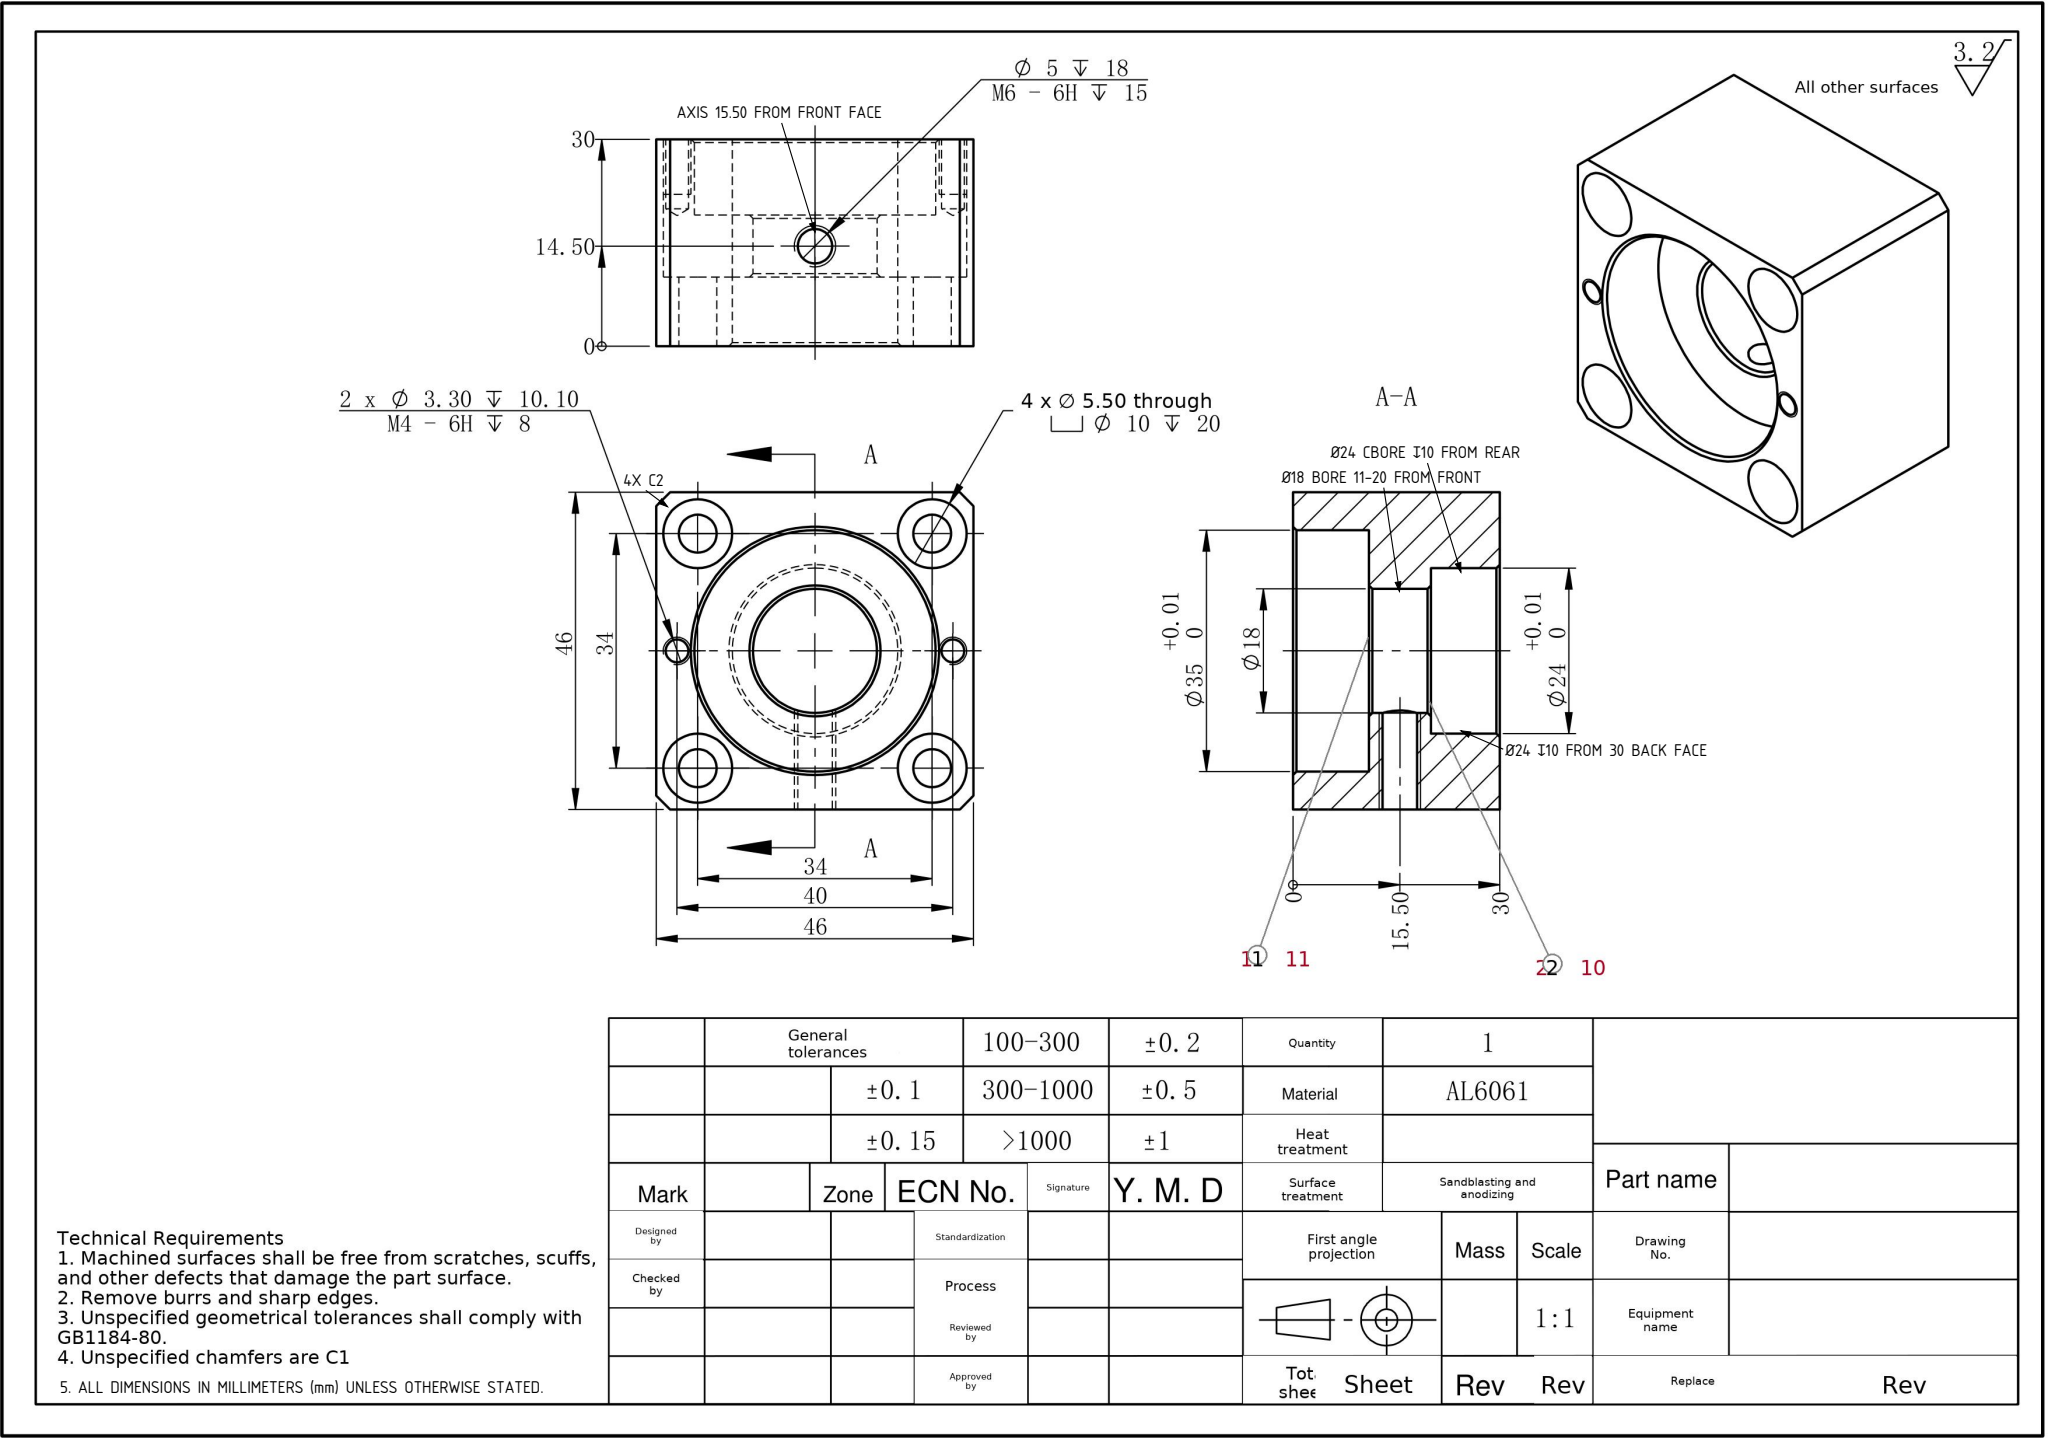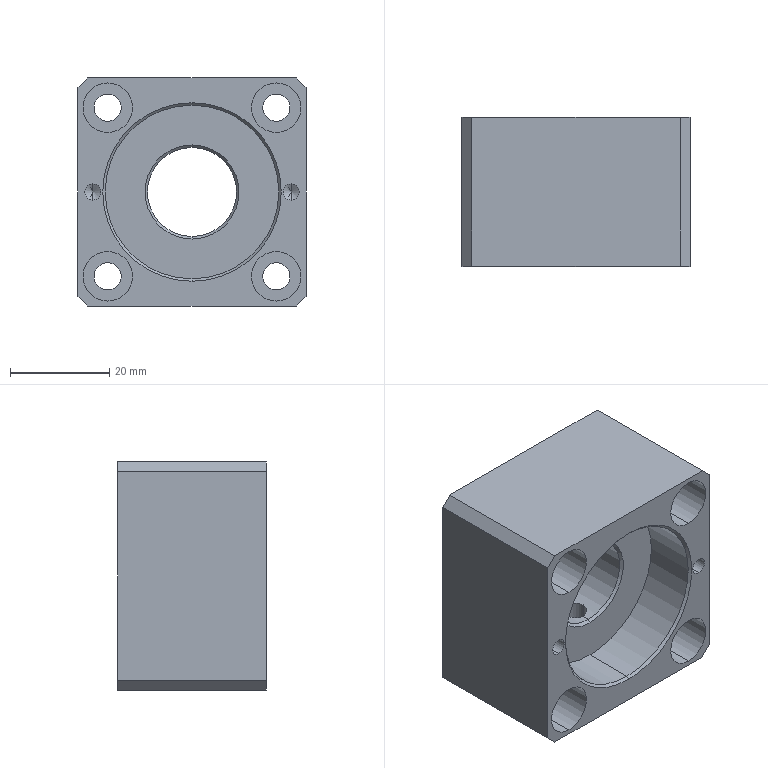Part | SolidWorks | mm | material AL6061 | 1 solid | 56 faces | box 46 x 30 x 46 mm | volume 38116 mm3 | cylinder 28 | plane 16 | cone 12 | commonest cylinder face diameters 10 x8 5.5 x8 3.3 x4 5 x2 35 x2 24 x2 18 x2
Drawing notes:
ALL DIMENSIONS IN MILLIMETERS (mm) UNLESS OTHERWISE STATED. | from the solid: STEP header units mm; bbox_xyz [46.0, 30.0, 46.0]
Ø18 THROUGH-BORE BETWEEN COUNTERBORES, SPANS 11 TO 20 FROM FRONT FACE (Y=0), AXIS AT X=23, Z=23. | from the solid: cylinders: hole/bore Ø18, axis y at [23,null,23], from 11.5 to 19.5 with 90° chamfers at both ends
Ø24 COUNTERBORE, DEPTH 10 FROM REAR FACE (Y=30), COAXIAL WITH Ø18 BORE. | from the solid: cylinders: hole/bore Ø24, axis y at [23,null,23], from 20.0 to 29.5 (0.5 chamfer at mouth)
4X CORNER CHAMFER C2 (2x2x45 DEG) FULL 30 HT, NOT C1 | from the solid: 4 inclined planes 45/90/45 deg, size 2.0 x 30.0 x 2.0 at bbox corners [0,0,0],[0,0,44],[44,0,0],[44,0,44]
M6 HOLE AXIS 15.50 FROM FRONT FACE (0); 14.50 IN TOP VIEW VOID | from the solid: Ø5 bore, axis Z, at [x=23, y=15.5], from z=0 to 14.4
A-A: Ø24 C'BORE DP 10 FROM 30 BACK FACE; '22' VOID | from the solid: Ø24 bore axis Y from y=20.0 to 30.0 (29.5 + 90 deg cone to face y=30), depth 10
build123d program:
from build123d import *

# Parameters (mm, degrees)
SKETCH1_W                                       = 46
SKETCH1_H                                       = 46
BOSS_EXTRUDE1_DEPTH                             = 15
SKETCH4_R                                       = 9
CUT_EXTRUDE1_DEPTH                              = 29
SKETCH5_R                                       = 12
CUT_EXTRUDE2_DEPTH                              = 10
CHAMFER1_SIZE                                   = 2
M5_HEX_SOCKET_HEAD_CAP_SCREW_CBORE1_D           = 5.5
M5_HEX_SOCKET_HEAD_CAP_SCREW_CBORE1_CBORE_D     = 10
M5_HEX_SOCKET_HEAD_CAP_SCREW_CBORE1_CBORE_DEPTH = 20
SKETCH8_R                                       = 17.5
CUT_EXTRUDE3_DEPTH                              = 11
CHAMFER2_SIZE                                   = 0.5
M6_TAPPED_HOLE1_D                               = 5
M6_TAPPED_HOLE1_DEPTH                           = 18
M6_TAPPED_HOLE1_TIP                             = 1.502
M4_TAPPED_HOLE1_D                               = 3.3
M4_TAPPED_HOLE1_DEPTH                           = 10.1
M4_TAPPED_HOLE1_TIP                             = 0.9914


with BuildPart() as part:
    # Sketch1 → Boss-Extrude1 (new, symmetric)
    with BuildSketch(Plane(origin=(0, 0, 0), x_dir=(1, 0, 0), z_dir=(0, 1, 0))):
        Rectangle(SKETCH1_W, SKETCH1_H)
    extrude(amount=BOSS_EXTRUDE1_DEPTH, both=True)

    # Sketch4 → Cut-Extrude1 (cut)
    with BuildSketch(Plane(origin=(0, 15, 0), x_dir=(1, 0, 0), z_dir=(0, 1, 0))):
        with Locations(Location((0, 0, 0), (0, 0, 270))):
            Circle(SKETCH4_R)
    extrude(amount=-CUT_EXTRUDE1_DEPTH, mode=Mode.SUBTRACT)

    # Sketch5 → Cut-Extrude2 (cut)
    with BuildSketch(Plane(origin=(0, 15, 0), x_dir=(1, 0, 0), z_dir=(0, 1, 0))):
        with Locations(Location((0, 0, 0), (0, 0, 270))):
            Circle(SKETCH5_R)
    extrude(amount=-CUT_EXTRUDE2_DEPTH, mode=Mode.SUBTRACT)

    # Chamfer1
    chamfer1_edges = [part.edges().sort_by_distance(p)[0] for p in [
        (23, 0, 23),
        (-23, 0, 23),
        (-23, 0, -23),
        (23, 0, -23),
    ]]
    chamfer(chamfer1_edges, length=CHAMFER1_SIZE)

    # M5 Hex Socket Head Cap Screw CBORE1 (through all)
    with Locations(Plane(origin=(0, -15, 0), x_dir=(-1, 0, 0), z_dir=(0, -1, 0))):
        with Locations((-17, -17), (17, -17), (17, 17), (-17, 17)):
            CounterBoreHole(M5_HEX_SOCKET_HEAD_CAP_SCREW_CBORE1_D / 2, M5_HEX_SOCKET_HEAD_CAP_SCREW_CBORE1_CBORE_D / 2, M5_HEX_SOCKET_HEAD_CAP_SCREW_CBORE1_CBORE_DEPTH)

    # Sketch8 → Cut-Extrude3 (cut)
    with BuildSketch(Plane.XZ.offset(15)):
        with Locations(Location((0, 0, 0), (0, 0, 270))):
            Circle(SKETCH8_R)
    extrude(amount=-CUT_EXTRUDE3_DEPTH, mode=Mode.SUBTRACT)

    # Chamfer2
    chamfer2_edges = [part.edges().sort_by_distance(p)[0] for p in [
        (0, 15, -12),
        (0, 5, -9),
        (0, -4, -9),
        (0, -15, 17.5),
    ]]
    chamfer(chamfer2_edges, length=CHAMFER2_SIZE)

    # M6 Tapped Hole1
    with Locations(Plane(origin=(0, 0, -23), x_dir=(-1, 0, 0), z_dir=(0, 0, -1))):
        with Locations((0, 0.5)):
            Hole(M6_TAPPED_HOLE1_D / 2, depth=M6_TAPPED_HOLE1_DEPTH)
            with Locations((0, 0, -(M6_TAPPED_HOLE1_DEPTH + M6_TAPPED_HOLE1_TIP / 2))):  # 118° drill point
                Cone(0, M6_TAPPED_HOLE1_D / 2, M6_TAPPED_HOLE1_TIP, mode=Mode.SUBTRACT)

    # M4 Tapped Hole1
    with Locations(Plane(origin=(0, -15, 0), x_dir=(-1, 0, 0), z_dir=(0, -1, 0))):
        with Locations((20, 0), (-20, 0)):
            Hole(M4_TAPPED_HOLE1_D / 2, depth=M4_TAPPED_HOLE1_DEPTH)
            with Locations((0, 0, -(M4_TAPPED_HOLE1_DEPTH + M4_TAPPED_HOLE1_TIP / 2))):  # 118° drill point
                Cone(0, M4_TAPPED_HOLE1_D / 2, M4_TAPPED_HOLE1_TIP, mode=Mode.SUBTRACT)


solid = part.part